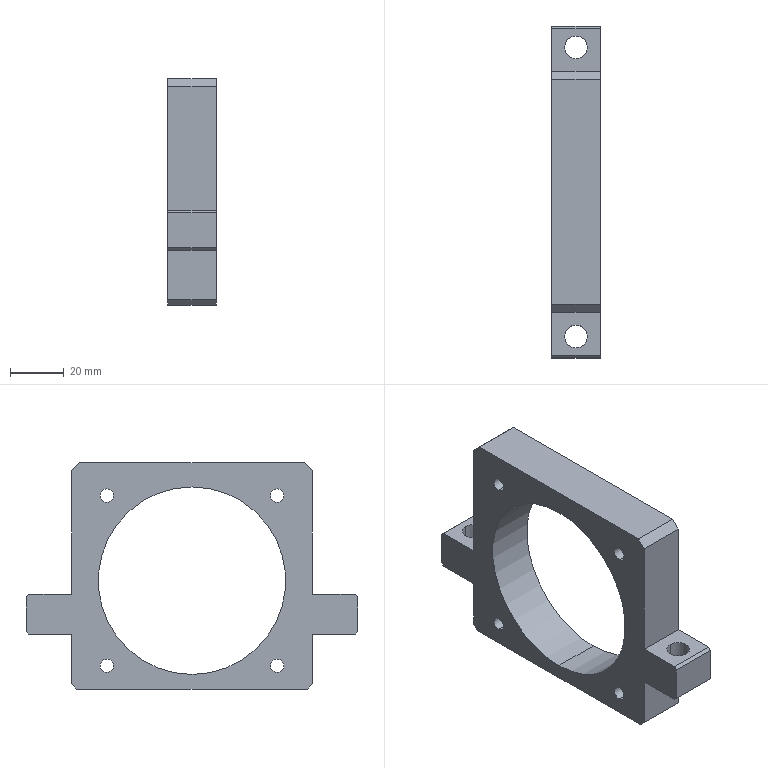Component | SolidWorks | 6G-TL06-Y-AxisMotorAssembly-2_6G-TL06.01.03-X-AxisMotorMountingPlate-1 | 1 solid | 36 faces | box 18 x 124 x 84.5 mm | volume 73412 mm3 | plane 22 | cylinder 14 | commonest cylinder face diameters 5 x8 8.5 x4 70 x2
build123d program:
from build123d import *

# Parameters (mm, degrees)
SKETCH1_2_W         = 84.5
SKETCH1_2_H         = 120
BOSS_EXTRUDE1_DEPTH = 18
SKETCH3_2_R         = 35
CUT_EXTRUDE2_DEPTH  = 76.558
M6_TAPPED_HOLE1_D   = 5
CUT_EXTRUDE3_DEPTH  = 76.558
CHAMFER3_SIZE       = 3
SKETCH7_R           = 3.25
CUT_EXTRUDE4_DEPTH  = 106.187
SKETCH3_W           = 25
SKETCH3_H           = 15
EXTRUDE1_DEPTH      = 76.558
SKETCH4_W           = 15
SKETCH4_H           = 17
EXTRUDE2_DEPTH      = 18
SKETCH5_R           = 4.25
EXTRUDE3_DEPTH      = 82.049
CHAMFER1_SIZE       = 2
CHAMFER2_SIZE       = 1


with BuildPart() as part:
    # Sketch1_2 → Boss-Extrude1 (new body)
    with BuildSketch(Plane.XY):
        Rectangle(SKETCH1_2_W, SKETCH1_2_H)
    extrude(amount=-BOSS_EXTRUDE1_DEPTH)

    # Sketch3_2 → Cut-Extrude2 (cut, through all)
    with BuildSketch(Plane.XY):
        with Locations((-1.75, 0)):
            Circle(SKETCH3_2_R)
    extrude(amount=-CUT_EXTRUDE2_DEPTH, mode=Mode.SUBTRACT)

    # M6 Tapped Hole1 (through all)
    with Locations(Plane.XY):
        with Locations((30.07, -31.82), (-33.57, -31.82), (-33.57, 31.82), (30.07, 31.82)):
            Hole(M6_TAPPED_HOLE1_D / 2)

    # Sketch6 → Cut-Extrude3 (cut, through all)
    with BuildSketch(Plane.XY):
        with BuildLine():
            Line((-26.5, 60), (42.25, 60))
            Line((42.25, 60), (42.25, 45))
            Line((42.25, 45), (-24.5, 45))
            ThreePointArc((-24.5, 45), (-25.914, 45.586), (-26.5, 47))
            Line((-26.5, 47), (-26.5, 60))
        make_face()
        with BuildLine():
            Line((42.25, -60), (42.25, -45))
            Line((42.25, -45), (-24.5, -45))
            ThreePointArc((-24.5, -45), (-25.914, -45.586), (-26.5, -47))
            Line((-26.5, -47), (-26.5, -60))
            Line((-26.5, -60), (42.25, -60))
        make_face()
    extrude(amount=-CUT_EXTRUDE3_DEPTH, mode=Mode.SUBTRACT)

    # Chamfer3
    chamfer3_edges = [part.edges().sort_by_distance(p)[0] for p in [
        (42.25, 45, -9),
        (42.25, -45, -9),
    ]]
    chamfer(chamfer3_edges, length=CHAMFER3_SIZE)

    # Sketch7 → Cut-Extrude4 (cut, through all)
    with BuildSketch(Plane.ZY.offset(42.25)):
        with Locations((-9, 53)):
            Circle(SKETCH7_R)
        with Locations(Location((-9, -53, 0), (0, 0, 270))):
            Circle(SKETCH7_R)
    extrude(amount=-CUT_EXTRUDE4_DEPTH, mode=Mode.SUBTRACT)

    # Sketch3 → Extrude1 (cut, through all)
    with BuildSketch(Plane(origin=(0, 0, -18), x_dir=(-1, 0, 0), z_dir=(0, 0, -1))):
        with Locations((29.75, 52.5)):
            Rectangle(SKETCH3_W, SKETCH3_H)
        with Locations((29.75, -52.5)):
            Rectangle(SKETCH3_W, SKETCH3_H)
    extrude(amount=-EXTRUDE1_DEPTH, mode=Mode.SUBTRACT)

    # Sketch4 → Extrude2 (add)
    with BuildSketch(Plane.XY):
        with Locations((-14.25, 53.5)):
            Rectangle(SKETCH4_W, SKETCH4_H)
        with Locations((-14.25, -53.5)):
            Rectangle(SKETCH4_W, SKETCH4_H)
    extrude(amount=-EXTRUDE2_DEPTH)

    # Sketch5 → Extrude3 (cut, through all)
    with BuildSketch(Plane(origin=(-6.75, 0, 0), x_dir=(0, 0, -1), z_dir=(1, 0, 0))):
        with Locations(Location((9, 54, 0), (0, 0, 90))):
            Circle(SKETCH5_R)
        with Locations(Location((9, -54, 0), (0, 0, 270))):
            Circle(SKETCH5_R)
    extrude(amount=-EXTRUDE3_DEPTH, mode=Mode.SUBTRACT)

    # Chamfer1
    chamfer1_edges = [part.edges().sort_by_distance(p)[0] for p in [
        (-42.25, 45, -9),
        (-42.25, -45, -9),
    ]]
    chamfer(chamfer1_edges, length=CHAMFER1_SIZE)

    # Chamfer2
    chamfer2_edges = [part.edges().sort_by_distance(p)[0] for p in [
        (-6.75, 62, -9),
        (-21.75, 62, -9),
        (-21.75, -62, -9),
        (-6.75, -62, -9),
    ]]
    chamfer(chamfer2_edges, length=CHAMFER2_SIZE)


solid = part.part

# Placed as in the assembly
solid = solid.moved(Location((182, 0, 21.75), (0, -90, 0)))